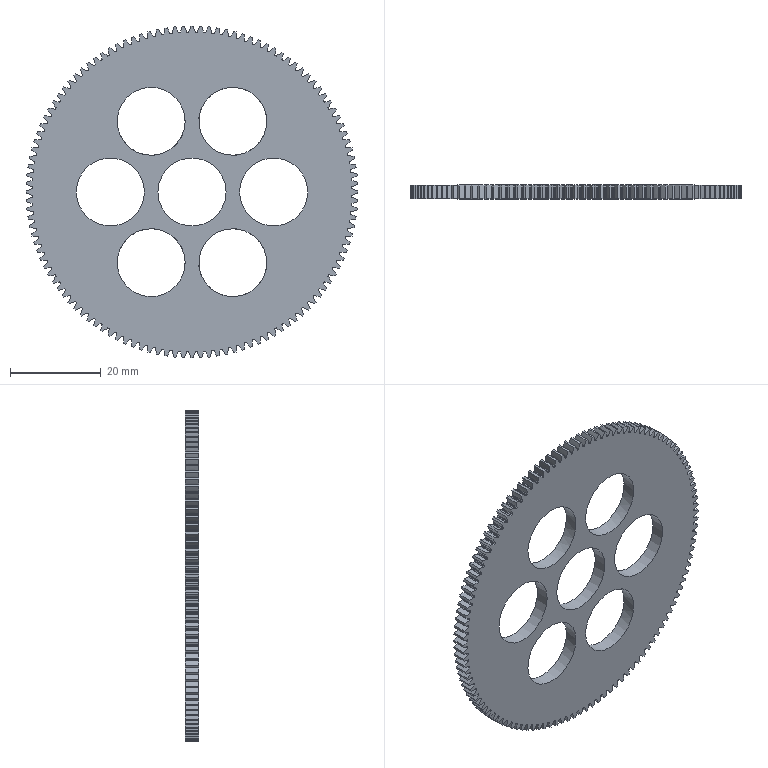Component | NX | 120_GEAR | 1 solid | 729 faces | volume 8478 mm3 | other 600 | cylinder 127 | plane 2 | commonest cylinder face diameters 70.5 x120 15 x7